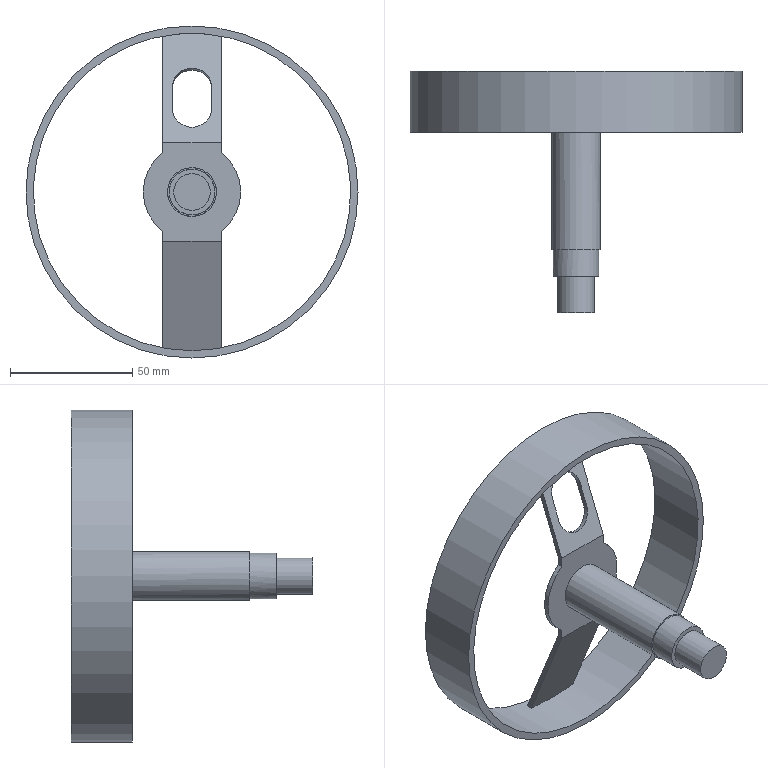Component | NX | 5 | 1 solid | 26 faces | volume 59281 mm3 | plane 17 | cylinder 9 | commonest cylinder face diameters 40 x2 16 x2 130 x1 136 x1 20 x1 18.782 x1 15 x1